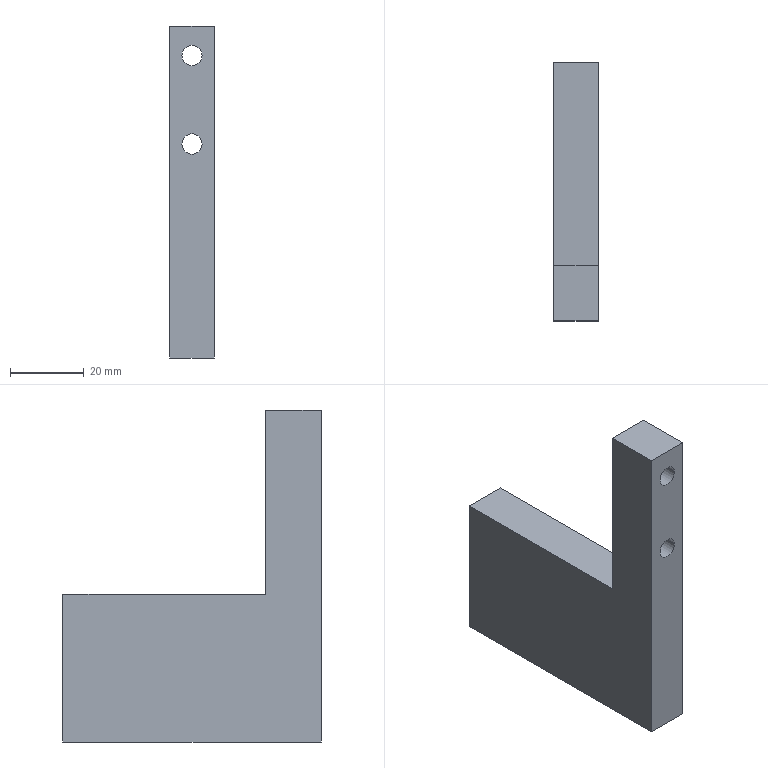Component | SolidWorks | CS021-A10-A026-1 | 1 solid | 16 faces | box 12 x 70 x 90 mm | volume 41682 mm3 | plane 8 | cylinder 6 | cone 2 | commonest cylinder face diameters 5.5 x4 4.2 x2 | material AL6061
build123d program:
from build123d import *

# Parameters (mm, degrees)
SKETCH1_W                  = 40
SKETCH1_H                  = 65
BOSS_EXTRUDE1_DEPTH        = 6
M5_TAPPED_HOLE1_D          = 4.2
M5_TAPPED_HOLE1_DEPTH      = 14.4
M5_TAPPED_HOLE1_TIP        = 1.262
SKETCH6_W                  = 90
SKETCH6_H                  = 15
BOSS_EXTRUDE2_DEPTH        = 12
F_5_5_5_5_DIAMETER_HOLE1_D = 5.5


with BuildPart() as part:
    # Sketch1 → Boss-Extrude1 (new, symmetric)
    with BuildSketch(Plane.XY):
        with Locations((20, 32.5)):
            Rectangle(SKETCH1_W, SKETCH1_H)
    extrude(amount=BOSS_EXTRUDE1_DEPTH, both=True)

    # M5 Tapped Hole1
    with Locations(Plane(origin=(0, 65, 0), x_dir=(1, 0, 0), z_dir=(0, 1, 0))):
        with Locations((20, 0)):
            Hole(M5_TAPPED_HOLE1_D / 2, depth=M5_TAPPED_HOLE1_DEPTH)
            with Locations((0, 0, -(M5_TAPPED_HOLE1_DEPTH + M5_TAPPED_HOLE1_TIP / 2))):  # 118° drill point
                Cone(0, M5_TAPPED_HOLE1_D / 2, M5_TAPPED_HOLE1_TIP, mode=Mode.SUBTRACT)

    # Sketch6 → Boss-Extrude2 (add)
    with BuildSketch(Plane.XY.offset(6)):
        with Locations((-5, 2.5)):
            Rectangle(SKETCH6_W, SKETCH6_H)
    extrude(amount=-BOSS_EXTRUDE2_DEPTH)

    # 5.5 _5.5_ Diameter Hole1 (through all)
    with Locations(Plane(origin=(0, 10, 0), x_dir=(1, 0, 0), z_dir=(0, 1, 0))):
        with Locations((-42, 0), (-18, 0)):
            Hole(F_5_5_5_5_DIAMETER_HOLE1_D / 2)


solid = part.part

# Placed as in the assembly
solid = solid.moved(Location((-7.551, 29.817, -65), (0, 90, 0)))
STEP:
#1=COLOUR_RGB('',0.7922,0.8196,0.9333);
#2=FILL_AREA_STYLE_COLOUR('',#1);
#3=FILL_AREA_STYLE('',(#2));
#4=SURFACE_STYLE_FILL_AREA(#3);
#5=SURFACE_SIDE_STYLE('',(#4));
#6=SURFACE_STYLE_USAGE(.BOTH.,#5);
#7=PRESENTATION_STYLE_ASSIGNMENT((#6));
#8=CARTESIAN_POINT('',(-0.4056,0.977,-0.9055));
#9=VERTEX_POINT('',#8);
#10=CARTESIAN_POINT('',(-0.189,0.977,-0.9055));
#11=VERTEX_POINT('',#10);
#12=CARTESIAN_POINT('',(-0.2973,0.977,-0.9055));
#13=DIRECTION('',(-0.,1.,0.));
#14=DIRECTION('',(1.,0.,0.));
#15=AXIS2_PLACEMENT_3D('',#12,#13,#14);
#16=CIRCLE('',#15,0.1083);
#17=EDGE_CURVE('',#9,#11,#16,.T.);
#18=ORIENTED_EDGE('',*,*,#17,.F.);
#19=CARTESIAN_POINT('',(-0.4056,1.568,-0.9055));
#20=VERTEX_POINT('',#19);
#21=CARTESIAN_POINT('',(-0.4056,1.568,-0.9055));
#22=DIRECTION('',(-0.,1.,0.));
#23=VECTOR('',#22,39.37);
#24=LINE('',#21,#23);
#25=EDGE_CURVE('',#9,#20,#24,.T.);
#26=ORIENTED_EDGE('',*,*,#25,.T.);
#27=CARTESIAN_POINT('',(-0.189,1.568,-0.9055));
#28=VERTEX_POINT('',#27);
#29=CARTESIAN_POINT('',(-0.2973,1.568,-0.9055));
#30=DIRECTION('',(-0.,1.,0.));
#31=DIRECTION('',(1.,0.,0.));
#32=AXIS2_PLACEMENT_3D('',#29,#30,#31);
#33=CIRCLE('',#32,0.1083);
#34=EDGE_CURVE('',#20,#28,#33,.T.);
#35=ORIENTED_EDGE('',*,*,#34,.T.);
#36=CARTESIAN_POINT('',(-0.189,1.568,-0.9055));
#37=DIRECTION('',(-0.,1.,0.));
#38=VECTOR('',#37,39.37);
#39=LINE('',#36,#38);
#40=EDGE_CURVE('',#11,#28,#39,.T.);
#41=ORIENTED_EDGE('',*,*,#40,.F.);
#42=EDGE_LOOP('',(#18,#26,#35,#41));
#43=FACE_OUTER_BOUND('',#42,.T.);
#44=CARTESIAN_POINT('',(-0.2973,1.568,-0.9055));
#45=DIRECTION('',(-0.,1.,0.));
#46=DIRECTION('',(1.,0.,0.));
#47=AXIS2_PLACEMENT_3D('',#44,#45,#46);
#48=CYLINDRICAL_SURFACE('',#47,0.1083);
#49=ADVANCED_FACE('',(#43),#48,.F.);
#50=CARTESIAN_POINT('',(-0.4056,0.977,-1.85));
#51=VERTEX_POINT('',#50);
#52=CARTESIAN_POINT('',(-0.189,0.977,-1.85));
#53=VERTEX_POINT('',#52);
#54=CARTESIAN_POINT('',(-0.2973,0.977,-1.85));
#55=DIRECTION('',(-0.,1.,0.));
#56=DIRECTION('',(1.,0.,0.));
#57=AXIS2_PLACEMENT_3D('',#54,#55,#56);
#58=CIRCLE('',#57,0.1083);
#59=EDGE_CURVE('',#51,#53,#58,.T.);
#60=ORIENTED_EDGE('',*,*,#59,.F.);
#61=CARTESIAN_POINT('',(-0.4056,1.568,-1.85));
#62=VERTEX_POINT('',#61);
#63=CARTESIAN_POINT('',(-0.4056,1.568,-1.85));
#64=DIRECTION('',(-0.,1.,0.));
#65=VECTOR('',#64,39.37);
#66=LINE('',#63,#65);
#67=EDGE_CURVE('',#51,#62,#66,.T.);
#68=ORIENTED_EDGE('',*,*,#67,.T.);
#69=CARTESIAN_POINT('',(-0.189,1.568,-1.85));
#70=VERTEX_POINT('',#69);
#71=CARTESIAN_POINT('',(-0.2973,1.568,-1.85));
#72=DIRECTION('',(-0.,1.,0.));
#73=DIRECTION('',(1.,0.,0.));
#74=AXIS2_PLACEMENT_3D('',#71,#72,#73);
#75=CIRCLE('',#74,0.1083);
#76=EDGE_CURVE('',#62,#70,#75,.T.);
#77=ORIENTED_EDGE('',*,*,#76,.T.);
#78=CARTESIAN_POINT('',(-0.189,1.568,-1.85));
#79=DIRECTION('',(-0.,1.,0.));
#80=VECTOR('',#79,39.37);
#81=LINE('',#78,#80);
#82=EDGE_CURVE('',#53,#70,#81,.T.);
#83=ORIENTED_EDGE('',*,*,#82,.F.);
#84=EDGE_LOOP('',(#60,#68,#77,#83));
#85=FACE_OUTER_BOUND('',#84,.T.);
#86=CARTESIAN_POINT('',(-0.2973,1.568,-1.85));
#87=DIRECTION('',(-0.,1.,0.));
#88=DIRECTION('',(1.,0.,0.));
#89=AXIS2_PLACEMENT_3D('',#86,#87,#88);
#90=CYLINDRICAL_SURFACE('',#89,0.1083);
#91=ADVANCED_FACE('',(#85),#90,.F.);
#92=CARTESIAN_POINT('',(-0.38,3.166,-3.346));
#93=VERTEX_POINT('',#92);
#94=CARTESIAN_POINT('',(-0.2146,3.166,-3.346));
#95=VERTEX_POINT('',#94);
#96=CARTESIAN_POINT('',(-0.2973,3.166,-3.346));
#97=DIRECTION('',(-0.,1.,0.));
#98=DIRECTION('',(1.,0.,0.));
#99=AXIS2_PLACEMENT_3D('',#96,#97,#98);
#100=CIRCLE('',#99,0.08268);
#101=EDGE_CURVE('',#93,#95,#100,.T.);
#102=ORIENTED_EDGE('',*,*,#101,.F.);
#103=CARTESIAN_POINT('',(-0.38,3.733,-3.346));
#104=VERTEX_POINT('',#103);
#105=CARTESIAN_POINT('',(-0.38,3.733,-3.346));
#106=DIRECTION('',(-0.,1.,0.));
#107=VECTOR('',#106,39.37);
#108=LINE('',#105,#107);
#109=EDGE_CURVE('',#93,#104,#108,.T.);
#110=ORIENTED_EDGE('',*,*,#109,.T.);
#111=CARTESIAN_POINT('',(-0.2146,3.733,-3.346));
#112=VERTEX_POINT('',#111);
#113=CARTESIAN_POINT('',(-0.2973,3.733,-3.346));
#114=DIRECTION('',(-0.,1.,0.));
#115=DIRECTION('',(1.,0.,0.));
#116=AXIS2_PLACEMENT_3D('',#113,#114,#115);
#117=CIRCLE('',#116,0.08268);
#118=EDGE_CURVE('',#104,#112,#117,.T.);
#119=ORIENTED_EDGE('',*,*,#118,.T.);
#120=CARTESIAN_POINT('',(-0.2146,3.733,-3.346));
#121=DIRECTION('',(-0.,1.,0.));
#122=VECTOR('',#121,39.37);
#123=LINE('',#120,#122);
#124=EDGE_CURVE('',#95,#112,#123,.T.);
#125=ORIENTED_EDGE('',*,*,#124,.F.);
#126=EDGE_LOOP('',(#102,#110,#119,#125));
#127=FACE_OUTER_BOUND('',#126,.T.);
#128=CARTESIAN_POINT('',(-0.2973,3.733,-3.346));
#129=DIRECTION('',(-0.,1.,0.));
#130=DIRECTION('',(1.,0.,0.));
#131=AXIS2_PLACEMENT_3D('',#128,#129,#130);
#132=CYLINDRICAL_SURFACE('',#131,0.08268);
#133=ADVANCED_FACE('',(#127),#132,.F.);
#134=CARTESIAN_POINT('',(-0.2973,3.116,-3.346));
#135=VERTEX_POINT('',#134);
#136=CARTESIAN_POINT('',(-0.2146,3.166,-3.346));
#137=DIRECTION('',(0.8572,0.515,0.));
#138=VECTOR('',#137,39.37);
#139=LINE('',#136,#138);
#140=EDGE_CURVE('',#135,#95,#139,.T.);
#141=ORIENTED_EDGE('',*,*,#140,.F.);
#142=CARTESIAN_POINT('',(-0.38,3.166,-3.346));
#143=DIRECTION('',(-0.8572,0.515,-0.));
#144=VECTOR('',#143,39.37);
#145=LINE('',#142,#144);
#146=EDGE_CURVE('',#135,#93,#145,.T.);
#147=ORIENTED_EDGE('',*,*,#146,.T.);
#148=ORIENTED_EDGE('',*,*,#101,.T.);
#149=EDGE_LOOP('',(#141,#147,#148));
#150=FACE_OUTER_BOUND('',#149,.T.);
#151=CARTESIAN_POINT('',(-0.2973,3.166,-3.346));
#152=DIRECTION('',(-0.,1.,0.));
#153=DIRECTION('',(1.,0.,0.));
#154=AXIS2_PLACEMENT_3D('',#151,#152,#153);
#155=CONICAL_SURFACE('',#154,0.08268,1.03);
#156=ADVANCED_FACE('',(#150),#155,.F.);
#157=CARTESIAN_POINT('',(-0.06108,3.733,-4.134));
#158=VERTEX_POINT('',#157);
#159=CARTESIAN_POINT('',(-0.5335,3.733,-4.134));
#160=VERTEX_POINT('',#159);
#161=CARTESIAN_POINT('',(-0.06108,3.733,-4.134));
#162=DIRECTION('',(-1.,0.,-0.));
#163=VECTOR('',#162,39.37);
#164=LINE('',#161,#163);
#165=EDGE_CURVE('',#158,#160,#164,.T.);
#166=ORIENTED_EDGE('',*,*,#165,.F.);
#167=CARTESIAN_POINT('',(-0.06108,0.977,-4.134));
#168=VERTEX_POINT('',#167);
#169=CARTESIAN_POINT('',(-0.06108,1.174,-4.134));
#170=DIRECTION('',(-0.,1.,0.));
#171=VECTOR('',#170,39.37);
#172=LINE('',#169,#171);
#173=EDGE_CURVE('',#168,#158,#172,.T.);
#174=ORIENTED_EDGE('',*,*,#173,.F.);
#175=CARTESIAN_POINT('',(-0.5335,0.977,-4.134));
#176=VERTEX_POINT('',#175);
#177=CARTESIAN_POINT('',(-0.5335,0.977,-4.134));
#178=DIRECTION('',(1.,-0.,0.));
#179=VECTOR('',#178,39.37);
#180=LINE('',#177,#179);
#181=EDGE_CURVE('',#176,#168,#180,.T.);
#182=ORIENTED_EDGE('',*,*,#181,.F.);
#183=CARTESIAN_POINT('',(-0.5335,1.174,-4.134));
#184=DIRECTION('',(-0.,1.,0.));
#185=VECTOR('',#184,39.37);
#186=LINE('',#183,#185);
#187=EDGE_CURVE('',#176,#160,#186,.T.);
#188=ORIENTED_EDGE('',*,*,#187,.T.);
#189=EDGE_LOOP('',(#166,#174,#182,#188));
#190=FACE_OUTER_BOUND('',#189,.T.);
#191=CARTESIAN_POINT('',(-0.06108,1.174,-4.134));
#192=DIRECTION('',(-0.,-0.,1.));
#193=DIRECTION('',(1.,-0.,0.));
#194=AXIS2_PLACEMENT_3D('',#191,#192,#193);
#195=PLANE('',#194);
#196=ADVANCED_FACE('',(#190),#195,.F.);
#197=CARTESIAN_POINT('',(-0.2973,3.733,-3.346));
#198=DIRECTION('',(-0.,1.,0.));
#199=DIRECTION('',(1.,0.,0.));
#200=AXIS2_PLACEMENT_3D('',#197,#198,#199);
#201=CIRCLE('',#200,0.08268);
#202=EDGE_CURVE('',#112,#104,#201,.T.);
#203=ORIENTED_EDGE('',*,*,#202,.F.);
#204=ORIENTED_EDGE('',*,*,#118,.F.);
#205=EDGE_LOOP('',(#203,#204));
#206=FACE_BOUND('',#205,.T.);
#207=CARTESIAN_POINT('',(-0.5335,3.733,-2.559));
#208=VERTEX_POINT('',#207);
#209=CARTESIAN_POINT('',(-0.5335,3.733,-2.559));
#210=DIRECTION('',(0.,0.,-1.));
#211=VECTOR('',#210,39.37);
#212=LINE('',#209,#211);
#213=EDGE_CURVE('',#208,#160,#212,.T.);
#214=ORIENTED_EDGE('',*,*,#213,.F.);
#215=CARTESIAN_POINT('',(-0.06108,3.733,-2.559));
#216=VERTEX_POINT('',#215);
#217=CARTESIAN_POINT('',(-0.06108,3.733,-2.559));
#218=DIRECTION('',(-1.,0.,-0.));
#219=VECTOR('',#218,39.37);
#220=LINE('',#217,#219);
#221=EDGE_CURVE('',#216,#208,#220,.T.);
#222=ORIENTED_EDGE('',*,*,#221,.F.);
#223=CARTESIAN_POINT('',(-0.06108,3.733,-2.559));
#224=DIRECTION('',(0.,0.,-1.));
#225=VECTOR('',#224,39.37);
#226=LINE('',#223,#225);
#227=EDGE_CURVE('',#216,#158,#226,.T.);
#228=ORIENTED_EDGE('',*,*,#227,.T.);
#229=ORIENTED_EDGE('',*,*,#165,.T.);
#230=EDGE_LOOP('',(#214,#222,#228,#229));
#231=FACE_OUTER_BOUND('',#230,.T.);
#232=CARTESIAN_POINT('',(-0.06108,3.733,-2.559));
#233=DIRECTION('',(0.,1.,0.));
#234=DIRECTION('',(1.,-0.,0.));
#235=AXIS2_PLACEMENT_3D('',#232,#233,#234);
#236=PLANE('',#235);
#237=ADVANCED_FACE('',(#206,#231),#236,.T.);
#238=CARTESIAN_POINT('',(-0.06108,1.568,-2.559));
#239=VERTEX_POINT('',#238);
#240=CARTESIAN_POINT('',(-0.5335,1.568,-2.559));
#241=VERTEX_POINT('',#240);
#242=CARTESIAN_POINT('',(-0.06108,1.568,-2.559));
#243=DIRECTION('',(-1.,0.,-0.));
#244=VECTOR('',#243,39.37);
#245=LINE('',#242,#244);
#246=EDGE_CURVE('',#239,#241,#245,.T.);
#247=ORIENTED_EDGE('',*,*,#246,.F.);
#248=CARTESIAN_POINT('',(-0.06108,1.174,-2.559));
#249=DIRECTION('',(-0.,1.,0.));
#250=VECTOR('',#249,39.37);
#251=LINE('',#248,#250);
#252=EDGE_CURVE('',#239,#216,#251,.T.);
#253=ORIENTED_EDGE('',*,*,#252,.T.);
#254=ORIENTED_EDGE('',*,*,#221,.T.);
#255=CARTESIAN_POINT('',(-0.5335,1.174,-2.559));
#256=DIRECTION('',(-0.,1.,0.));
#257=VECTOR('',#256,39.37);
#258=LINE('',#255,#257);
#259=EDGE_CURVE('',#241,#208,#258,.T.);
#260=ORIENTED_EDGE('',*,*,#259,.F.);
#261=EDGE_LOOP('',(#247,#253,#254,#260));
#262=FACE_OUTER_BOUND('',#261,.T.);
#263=CARTESIAN_POINT('',(-0.06108,1.174,-2.559));
#264=DIRECTION('',(-0.,-0.,1.));
#265=DIRECTION('',(1.,-0.,0.));
#266=AXIS2_PLACEMENT_3D('',#263,#264,#265);
#267=PLANE('',#266);
#268=ADVANCED_FACE('',(#262),#267,.T.);
#269=CARTESIAN_POINT('',(-0.06108,0.977,-0.5906));
#270=VERTEX_POINT('',#269);
#271=CARTESIAN_POINT('',(-0.06108,0.977,-4.134));
#272=DIRECTION('',(0.,0.,-1.));
#273=VECTOR('',#272,39.37);
#274=LINE('',#271,#273);
#275=EDGE_CURVE('',#270,#168,#274,.T.);
#276=ORIENTED_EDGE('',*,*,#275,.T.);
#277=ORIENTED_EDGE('',*,*,#173,.T.);
#278=ORIENTED_EDGE('',*,*,#227,.F.);
#279=ORIENTED_EDGE('',*,*,#252,.F.);
#280=CARTESIAN_POINT('',(-0.06108,1.568,-0.5906));
#281=VERTEX_POINT('',#280);
#282=CARTESIAN_POINT('',(-0.06108,1.568,-4.134));
#283=DIRECTION('',(-0.,-0.,1.));
#284=VECTOR('',#283,39.37);
#285=LINE('',#282,#284);
#286=EDGE_CURVE('',#239,#281,#285,.T.);
#287=ORIENTED_EDGE('',*,*,#286,.T.);
#288=CARTESIAN_POINT('',(-0.06108,1.568,-0.5906));
#289=DIRECTION('',(0.,-1.,-0.));
#290=VECTOR('',#289,39.37);
#291=LINE('',#288,#290);
#292=EDGE_CURVE('',#281,#270,#291,.T.);
#293=ORIENTED_EDGE('',*,*,#292,.T.);
#294=EDGE_LOOP('',(#276,#277,#278,#279,#287,#293));
#295=FACE_OUTER_BOUND('',#294,.T.);
#296=CARTESIAN_POINT('',(-0.06108,1.174,-2.559));
#297=DIRECTION('',(1.,-0.,0.));
#298=DIRECTION('',(0.,0.,-1.));
#299=AXIS2_PLACEMENT_3D('',#296,#297,#298);
#300=PLANE('',#299);
#301=ADVANCED_FACE('',(#295),#300,.T.);
#302=ORIENTED_EDGE('',*,*,#187,.F.);
#303=CARTESIAN_POINT('',(-0.5335,0.977,-0.5906));
#304=VERTEX_POINT('',#303);
#305=CARTESIAN_POINT('',(-0.5335,0.977,-4.134));
#306=DIRECTION('',(0.,0.,-1.));
#307=VECTOR('',#306,39.37);
#308=LINE('',#305,#307);
#309=EDGE_CURVE('',#304,#176,#308,.T.);
#310=ORIENTED_EDGE('',*,*,#309,.F.);
#311=CARTESIAN_POINT('',(-0.5335,1.568,-0.5906));
#312=VERTEX_POINT('',#311);
#313=CARTESIAN_POINT('',(-0.5335,1.568,-0.5906));
#314=DIRECTION('',(0.,-1.,-0.));
#315=VECTOR('',#314,39.37);
#316=LINE('',#313,#315);
#317=EDGE_CURVE('',#312,#304,#316,.T.);
#318=ORIENTED_EDGE('',*,*,#317,.F.);
#319=CARTESIAN_POINT('',(-0.5335,1.568,-4.134));
#320=DIRECTION('',(-0.,-0.,1.));
#321=VECTOR('',#320,39.37);
#322=LINE('',#319,#321);
#323=EDGE_CURVE('',#241,#312,#322,.T.);
#324=ORIENTED_EDGE('',*,*,#323,.F.);
#325=ORIENTED_EDGE('',*,*,#259,.T.);
#326=ORIENTED_EDGE('',*,*,#213,.T.);
#327=EDGE_LOOP('',(#302,#310,#318,#324,#325,#326));
#328=FACE_OUTER_BOUND('',#327,.T.);
#329=CARTESIAN_POINT('',(-0.5335,1.174,-2.559));
#330=DIRECTION('',(1.,-0.,0.));
#331=DIRECTION('',(0.,0.,-1.));
#332=AXIS2_PLACEMENT_3D('',#329,#330,#331);
#333=PLANE('',#332);
#334=ADVANCED_FACE('',(#328),#333,.F.);
#335=ORIENTED_EDGE('',*,*,#146,.F.);
#336=ORIENTED_EDGE('',*,*,#140,.T.);
#337=CARTESIAN_POINT('',(-0.2973,3.166,-3.346));
#338=DIRECTION('',(-0.,1.,0.));
#339=DIRECTION('',(1.,0.,0.));
#340=AXIS2_PLACEMENT_3D('',#337,#338,#339);
#341=CIRCLE('',#340,0.08268);
#342=EDGE_CURVE('',#95,#93,#341,.T.);
#343=ORIENTED_EDGE('',*,*,#342,.T.);
#344=EDGE_LOOP('',(#335,#336,#343));
#345=FACE_OUTER_BOUND('',#344,.T.);
#346=CARTESIAN_POINT('',(-0.2973,3.166,-3.346));
#347=DIRECTION('',(-0.,1.,0.));
#348=DIRECTION('',(1.,0.,0.));
#349=AXIS2_PLACEMENT_3D('',#346,#347,#348);
#350=CONICAL_SURFACE('',#349,0.08268,1.03);
#351=ADVANCED_FACE('',(#345),#350,.F.);
#352=ORIENTED_EDGE('',*,*,#109,.F.);
#353=ORIENTED_EDGE('',*,*,#342,.F.);
#354=ORIENTED_EDGE('',*,*,#124,.T.);
#355=ORIENTED_EDGE('',*,*,#202,.T.);
#356=EDGE_LOOP('',(#352,#353,#354,#355));
#357=FACE_OUTER_BOUND('',#356,.T.);
#358=CARTESIAN_POINT('',(-0.2973,3.733,-3.346));
#359=DIRECTION('',(-0.,1.,0.));
#360=DIRECTION('',(1.,0.,0.));
#361=AXIS2_PLACEMENT_3D('',#358,#359,#360);
#362=CYLINDRICAL_SURFACE('',#361,0.08268);
#363=ADVANCED_FACE('',(#357),#362,.F.);
#364=CARTESIAN_POINT('',(-0.2973,0.977,-0.9055));
#365=DIRECTION('',(-0.,1.,0.));
#366=DIRECTION('',(1.,0.,0.));
#367=AXIS2_PLACEMENT_3D('',#364,#365,#366);
#368=CIRCLE('',#367,0.1083);
#369=EDGE_CURVE('',#11,#9,#368,.T.);
#370=ORIENTED_EDGE('',*,*,#369,.T.);
#371=ORIENTED_EDGE('',*,*,#17,.T.);
#372=EDGE_LOOP('',(#370,#371));
#373=FACE_BOUND('',#372,.T.);
#374=CARTESIAN_POINT('',(-0.2973,0.977,-1.85));
#375=DIRECTION('',(-0.,1.,0.));
#376=DIRECTION('',(1.,0.,0.));
#377=AXIS2_PLACEMENT_3D('',#374,#375,#376);
#378=CIRCLE('',#377,0.1083);
#379=EDGE_CURVE('',#53,#51,#378,.T.);
#380=ORIENTED_EDGE('',*,*,#379,.T.);
#381=ORIENTED_EDGE('',*,*,#59,.T.);
#382=EDGE_LOOP('',(#380,#381));
#383=FACE_BOUND('',#382,.T.);
#384=ORIENTED_EDGE('',*,*,#275,.F.);
#385=CARTESIAN_POINT('',(-0.5335,0.977,-0.5906));
#386=DIRECTION('',(1.,-0.,0.));
#387=VECTOR('',#386,39.37);
#388=LINE('',#385,#387);
#389=EDGE_CURVE('',#304,#270,#388,.T.);
#390=ORIENTED_EDGE('',*,*,#389,.F.);
#391=ORIENTED_EDGE('',*,*,#309,.T.);
#392=ORIENTED_EDGE('',*,*,#181,.T.);
#393=EDGE_LOOP('',(#384,#390,#391,#392));
#394=FACE_OUTER_BOUND('',#393,.T.);
#395=CARTESIAN_POINT('',(-0.5335,0.977,-4.134));
#396=DIRECTION('',(0.,-1.,-0.));
#397=DIRECTION('',(0.,0.,-1.));
#398=AXIS2_PLACEMENT_3D('',#395,#396,#397);
#399=PLANE('',#398);
#400=ADVANCED_FACE('',(#373,#383,#394),#399,.T.);
#401=ORIENTED_EDGE('',*,*,#292,.F.);
#402=CARTESIAN_POINT('',(-0.5335,1.568,-0.5906));
#403=DIRECTION('',(1.,-0.,0.));
#404=VECTOR('',#403,39.37);
#405=LINE('',#402,#404);
#406=EDGE_CURVE('',#312,#281,#405,.T.);
#407=ORIENTED_EDGE('',*,*,#406,.F.);
#408=ORIENTED_EDGE('',*,*,#317,.T.);
#409=ORIENTED_EDGE('',*,*,#389,.T.);
#410=EDGE_LOOP('',(#401,#407,#408,#409));
#411=FACE_OUTER_BOUND('',#410,.T.);
#412=CARTESIAN_POINT('',(-0.5335,1.568,-0.5906));
#413=DIRECTION('',(-0.,-0.,1.));
#414=DIRECTION('',(0.,-1.,-0.));
#415=AXIS2_PLACEMENT_3D('',#412,#413,#414);
#416=PLANE('',#415);
#417=ADVANCED_FACE('',(#411),#416,.T.);
#418=CARTESIAN_POINT('',(-0.2973,1.568,-0.9055));
#419=DIRECTION('',(-0.,1.,0.));
#420=DIRECTION('',(1.,0.,0.));
#421=AXIS2_PLACEMENT_3D('',#418,#419,#420);
#422=CIRCLE('',#421,0.1083);
#423=EDGE_CURVE('',#28,#20,#422,.T.);
#424=ORIENTED_EDGE('',*,*,#423,.F.);
#425=ORIENTED_EDGE('',*,*,#34,.F.);
#426=EDGE_LOOP('',(#424,#425));
#427=FACE_BOUND('',#426,.T.);
#428=CARTESIAN_POINT('',(-0.2973,1.568,-1.85));
#429=DIRECTION('',(-0.,1.,0.));
#430=DIRECTION('',(1.,0.,0.));
#431=AXIS2_PLACEMENT_3D('',#428,#429,#430);
#432=CIRCLE('',#431,0.1083);
#433=EDGE_CURVE('',#70,#62,#432,.T.);
#434=ORIENTED_EDGE('',*,*,#433,.F.);
#435=ORIENTED_EDGE('',*,*,#76,.F.);
#436=EDGE_LOOP('',(#434,#435));
#437=FACE_BOUND('',#436,.T.);
#438=ORIENTED_EDGE('',*,*,#286,.F.);
#439=ORIENTED_EDGE('',*,*,#246,.T.);
#440=ORIENTED_EDGE('',*,*,#323,.T.);
#441=ORIENTED_EDGE('',*,*,#406,.T.);
#442=EDGE_LOOP('',(#438,#439,#440,#441));
#443=FACE_OUTER_BOUND('',#442,.T.);
#444=CARTESIAN_POINT('',(-0.5335,1.568,-4.134));
#445=DIRECTION('',(-0.,1.,0.));
#446=DIRECTION('',(-0.,-0.,1.));
#447=AXIS2_PLACEMENT_3D('',#444,#445,#446);
#448=PLANE('',#447);
#449=ADVANCED_FACE('',(#427,#437,#443),#448,.T.);
#450=ORIENTED_EDGE('',*,*,#67,.F.);
#451=ORIENTED_EDGE('',*,*,#379,.F.);
#452=ORIENTED_EDGE('',*,*,#82,.T.);
#453=ORIENTED_EDGE('',*,*,#433,.T.);
#454=EDGE_LOOP('',(#450,#451,#452,#453));
#455=FACE_OUTER_BOUND('',#454,.T.);
#456=CARTESIAN_POINT('',(-0.2973,1.568,-1.85));
#457=DIRECTION('',(-0.,1.,0.));
#458=DIRECTION('',(1.,0.,0.));
#459=AXIS2_PLACEMENT_3D('',#456,#457,#458);
#460=CYLINDRICAL_SURFACE('',#459,0.1083);
#461=ADVANCED_FACE('',(#455),#460,.F.);
#462=ORIENTED_EDGE('',*,*,#25,.F.);
#463=ORIENTED_EDGE('',*,*,#369,.F.);
#464=ORIENTED_EDGE('',*,*,#40,.T.);
#465=ORIENTED_EDGE('',*,*,#423,.T.);
#466=EDGE_LOOP('',(#462,#463,#464,#465));
#467=FACE_OUTER_BOUND('',#466,.T.);
#468=CARTESIAN_POINT('',(-0.2973,1.568,-0.9055));
#469=DIRECTION('',(-0.,1.,0.));
#470=DIRECTION('',(1.,0.,0.));
#471=AXIS2_PLACEMENT_3D('',#468,#469,#470);
#472=CYLINDRICAL_SURFACE('',#471,0.1083);
#473=ADVANCED_FACE('',(#467),#472,.F.);
#474=CLOSED_SHELL('',(#49,#91,#133,#156,#196,#237,#268,#301,#334,#351,#363,#400,#417,#449,#461,#473));
#475=MANIFOLD_SOLID_BREP('',#474);
#476=STYLED_ITEM('',(#7),#475);
#477=(LENGTH_UNIT()NAMED_UNIT(*)SI_UNIT($,.METRE.));
#478=LENGTH_MEASURE_WITH_UNIT(LENGTH_MEASURE(0.0254),#477);
#479=DIMENSIONAL_EXPONENTS(1.,0.,0.,0.,0.,0.,0.);
#480=(CONVERSION_BASED_UNIT('',#478)LENGTH_UNIT()NAMED_UNIT(#479));
#481=UNCERTAINTY_MEASURE_WITH_UNIT(LENGTH_MEASURE(0.00001),#480,'','');
#482=(NAMED_UNIT(*)PLANE_ANGLE_UNIT()SI_UNIT($,.RADIAN.));
#483=(NAMED_UNIT(*)SI_UNIT($,.STERADIAN.)SOLID_ANGLE_UNIT());
#484=(GEOMETRIC_REPRESENTATION_CONTEXT(3)GLOBAL_UNCERTAINTY_ASSIGNED_CONTEXT((#481))GLOBAL_UNIT_ASSIGNED_CONTEXT((#480,#482,#483))REPRESENTATION_CONTEXT('',''));
#485=MECHANICAL_DESIGN_GEOMETRIC_PRESENTATION_REPRESENTATION('',(#476),#484);
#486=CARTESIAN_POINT('',(0.,0.,0.));
#487=DIRECTION('',(0.,0.,1.));
#488=DIRECTION('',(1.,0.,0.));
#489=AXIS2_PLACEMENT_3D('',#486,#487,#488);
#490=(LENGTH_UNIT()NAMED_UNIT(*)SI_UNIT($,.METRE.));
#491=LENGTH_MEASURE_WITH_UNIT(LENGTH_MEASURE(0.0254),#490);
#492=DIMENSIONAL_EXPONENTS(1.,0.,0.,0.,0.,0.,0.);
#493=(CONVERSION_BASED_UNIT('',#491)LENGTH_UNIT()NAMED_UNIT(#492));
#494=UNCERTAINTY_MEASURE_WITH_UNIT(LENGTH_MEASURE(0.00001),#493,'','');
#495=(NAMED_UNIT(*)PLANE_ANGLE_UNIT()SI_UNIT($,.RADIAN.));
#496=(NAMED_UNIT(*)SI_UNIT($,.STERADIAN.)SOLID_ANGLE_UNIT());
#497=(GEOMETRIC_REPRESENTATION_CONTEXT(3)GLOBAL_UNCERTAINTY_ASSIGNED_CONTEXT((#494))GLOBAL_UNIT_ASSIGNED_CONTEXT((#493,#495,#496))REPRESENTATION_CONTEXT('',''));
#498=ADVANCED_BREP_SHAPE_REPRESENTATION('',(#475,#489),#497);
#499=PRESENTATION_LAYER_ASSIGNMENT('','',(#476));